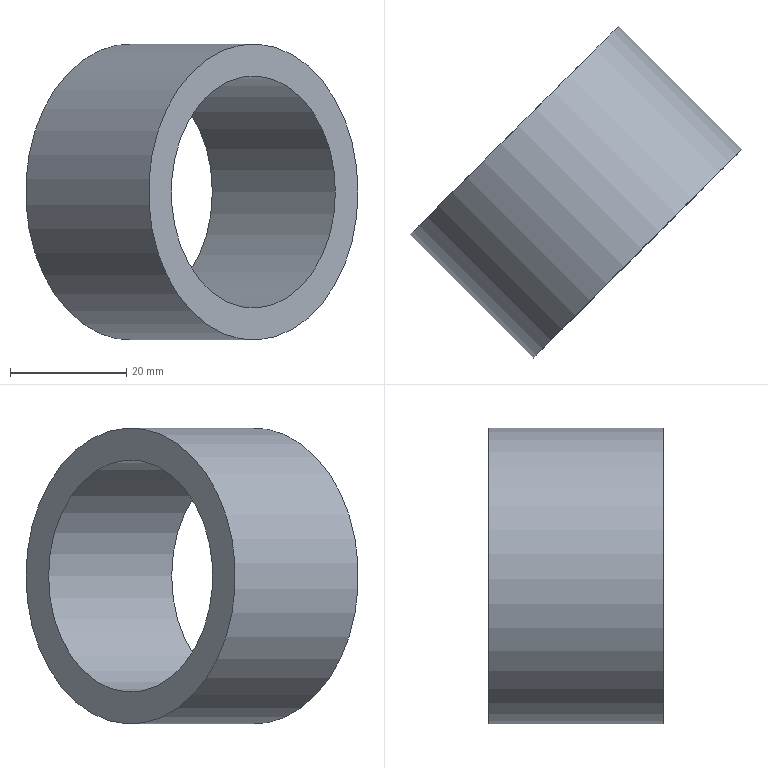Component | NX | CONN_FRAME_CONN_POST | 1 solid | 4 faces | box 57.28 x 57.28 x 51 mm | volume 23586 mm3 | cylinder 2 | plane 2 | commonest cylinder face diameters 51 x1 40 x1
STEP:
#1=CARTESIAN_POINT('',(0.,0.,0.));
#2=DIRECTION('',(0.,0.,1.));
#3=DIRECTION('',(1.,0.,0.));
#4=AXIS2_PLACEMENT_3D('',#1,#2,#3);
#5=CARTESIAN_POINT('',(-329.579,372.087,460.));
#6=VERTEX_POINT('',#5);
#7=CARTESIAN_POINT('',(-347.61,354.056,460.));
#8=DIRECTION('',(0.7071,-0.7071,0.));
#9=DIRECTION('',(0.7071,0.7071,0.));
#10=AXIS2_PLACEMENT_3D('',#7,#8,#9);
#11=CIRCLE('',#10,25.5);
#12=CARTESIAN_POINT('',(-347.61,354.056,460.));
#13=DIRECTION('',(0.7071,-0.7071,0.));
#14=DIRECTION('',(-0.7071,-0.7071,0.));
#15=AXIS2_PLACEMENT_3D('',#12,#13,#14);
#16=CYLINDRICAL_SURFACE('',#15,25.5);
#17=CARTESIAN_POINT('',(3.142,0.));
#18=DIRECTION('',(1.,0.));
#19=VECTOR('',#18,1.);
#20=LINE('',#17,#19);
#21=(GEOMETRIC_REPRESENTATION_CONTEXT(2)PARAMETRIC_REPRESENTATION_CONTEXT()REPRESENTATION_CONTEXT('',''));
#22=DEFINITIONAL_REPRESENTATION('',(#20),#21);
#23=PCURVE('',#16,#22);
#24=CARTESIAN_POINT('',(-347.61,354.056,460.));
#25=DIRECTION('',(0.7071,-0.7071,0.));
#26=DIRECTION('',(-0.7071,-0.7071,0.));
#27=AXIS2_PLACEMENT_3D('',#24,#25,#26);
#28=PLANE('',#27);
#29=CARTESIAN_POINT('',(0.,0.));
#30=DIRECTION('',(-1.,0.));
#31=AXIS2_PLACEMENT_2D('',#29,#30);
#32=CIRCLE('',#31,25.5);
#33=(GEOMETRIC_REPRESENTATION_CONTEXT(2)PARAMETRIC_REPRESENTATION_CONTEXT()REPRESENTATION_CONTEXT('',''));
#34=DEFINITIONAL_REPRESENTATION('',(#32),#33);
#35=PCURVE('',#28,#34);
#36=SURFACE_CURVE('',#11,(#23,#35),.PCURVE_S1.);
#37=EDGE_CURVE('',#6,#6,#36,.T.);
#38=ORIENTED_EDGE('',*,*,#37,.T.);
#39=CARTESIAN_POINT('',(-308.366,350.874,460.));
#40=VERTEX_POINT('',#39);
#41=CARTESIAN_POINT('',(-329.579,372.087,460.));
#42=CARTESIAN_POINT('',(-308.366,350.874,460.));
#43=B_SPLINE_CURVE_WITH_KNOTS('',1,(#41,#42),.UNSPECIFIED.,.F.,.F.,(2,2),(0.,30.),.PIECEWISE_BEZIER_KNOTS.);
#44=CARTESIAN_POINT('',(9.425,0.));
#45=DIRECTION('',(0.,1.));
#46=VECTOR('',#45,1.);
#47=LINE('',#44,#46);
#48=(GEOMETRIC_REPRESENTATION_CONTEXT(2)PARAMETRIC_REPRESENTATION_CONTEXT()REPRESENTATION_CONTEXT('',''));
#49=DEFINITIONAL_REPRESENTATION('',(#47),#48);
#50=PCURVE('',#16,#49);
#51=CARTESIAN_POINT('',(3.142,0.));
#52=DIRECTION('',(0.,1.));
#53=VECTOR('',#52,1.);
#54=LINE('',#51,#53);
#55=(GEOMETRIC_REPRESENTATION_CONTEXT(2)PARAMETRIC_REPRESENTATION_CONTEXT()REPRESENTATION_CONTEXT('',''));
#56=DEFINITIONAL_REPRESENTATION('',(#54),#55);
#57=PCURVE('',#16,#56);
#58=SEAM_CURVE('',#43,(#50,#57),.PCURVE_S1.);
#59=EDGE_CURVE('',#6,#40,#58,.T.);
#60=ORIENTED_EDGE('',*,*,#59,.T.);
#61=CARTESIAN_POINT('',(-326.397,332.843,460.));
#62=DIRECTION('',(0.7071,-0.7071,0.));
#63=DIRECTION('',(0.7071,0.7071,0.));
#64=AXIS2_PLACEMENT_3D('',#61,#62,#63);
#65=CIRCLE('',#64,25.5);
#66=CARTESIAN_POINT('',(3.142,30.));
#67=DIRECTION('',(1.,0.));
#68=VECTOR('',#67,1.);
#69=LINE('',#66,#68);
#70=(GEOMETRIC_REPRESENTATION_CONTEXT(2)PARAMETRIC_REPRESENTATION_CONTEXT()REPRESENTATION_CONTEXT('',''));
#71=DEFINITIONAL_REPRESENTATION('',(#69),#70);
#72=PCURVE('',#16,#71);
#73=CARTESIAN_POINT('',(-326.397,332.843,460.));
#74=DIRECTION('',(0.7071,-0.7071,0.));
#75=DIRECTION('',(-0.7071,-0.7071,0.));
#76=AXIS2_PLACEMENT_3D('',#73,#74,#75);
#77=PLANE('',#76);
#78=CARTESIAN_POINT('',(0.,0.));
#79=DIRECTION('',(-1.,0.));
#80=AXIS2_PLACEMENT_2D('',#78,#79);
#81=CIRCLE('',#80,25.5);
#82=(GEOMETRIC_REPRESENTATION_CONTEXT(2)PARAMETRIC_REPRESENTATION_CONTEXT()REPRESENTATION_CONTEXT('',''));
#83=DEFINITIONAL_REPRESENTATION('',(#81),#82);
#84=PCURVE('',#77,#83);
#85=SURFACE_CURVE('',#65,(#72,#84),.PCURVE_S1.);
#86=EDGE_CURVE('',#40,#40,#85,.T.);
#87=ORIENTED_EDGE('',*,*,#86,.F.);
#88=ORIENTED_EDGE('',*,*,#59,.F.);
#89=EDGE_LOOP('',(#38,#60,#87,#88));
#90=FACE_BOUND('',#89,.T.);
#91=ADVANCED_FACE('',(#90),#16,.T.);
#92=CARTESIAN_POINT('',(-333.468,368.198,460.));
#93=VERTEX_POINT('',#92);
#94=CARTESIAN_POINT('',(-347.61,354.056,460.));
#95=DIRECTION('',(0.7071,-0.7071,0.));
#96=DIRECTION('',(0.7071,0.7071,0.));
#97=AXIS2_PLACEMENT_3D('',#94,#95,#96);
#98=CIRCLE('',#97,20.);
#99=CARTESIAN_POINT('',(-347.61,354.056,460.));
#100=DIRECTION('',(0.7071,-0.7071,0.));
#101=DIRECTION('',(-0.7071,-0.7071,0.));
#102=AXIS2_PLACEMENT_3D('',#99,#100,#101);
#103=CYLINDRICAL_SURFACE('',#102,20.);
#104=CARTESIAN_POINT('',(3.142,0.));
#105=DIRECTION('',(1.,0.));
#106=VECTOR('',#105,1.);
#107=LINE('',#104,#106);
#108=(GEOMETRIC_REPRESENTATION_CONTEXT(2)PARAMETRIC_REPRESENTATION_CONTEXT()REPRESENTATION_CONTEXT('',''));
#109=DEFINITIONAL_REPRESENTATION('',(#107),#108);
#110=PCURVE('',#103,#109);
#111=CARTESIAN_POINT('',(0.,0.));
#112=DIRECTION('',(-1.,0.));
#113=AXIS2_PLACEMENT_2D('',#111,#112);
#114=CIRCLE('',#113,20.);
#115=(GEOMETRIC_REPRESENTATION_CONTEXT(2)PARAMETRIC_REPRESENTATION_CONTEXT()REPRESENTATION_CONTEXT('',''));
#116=DEFINITIONAL_REPRESENTATION('',(#114),#115);
#117=PCURVE('',#28,#116);
#118=SURFACE_CURVE('',#98,(#110,#117),.PCURVE_S1.);
#119=EDGE_CURVE('',#93,#93,#118,.T.);
#120=ORIENTED_EDGE('',*,*,#119,.T.);
#121=CARTESIAN_POINT('',(-312.255,346.985,460.));
#122=VERTEX_POINT('',#121);
#123=CARTESIAN_POINT('',(-333.468,368.198,460.));
#124=CARTESIAN_POINT('',(-312.255,346.985,460.));
#125=B_SPLINE_CURVE_WITH_KNOTS('',1,(#123,#124),.UNSPECIFIED.,.F.,.F.,(2,2),(0.,30.),.PIECEWISE_BEZIER_KNOTS.);
#126=CARTESIAN_POINT('',(9.425,0.));
#127=DIRECTION('',(0.,1.));
#128=VECTOR('',#127,1.);
#129=LINE('',#126,#128);
#130=(GEOMETRIC_REPRESENTATION_CONTEXT(2)PARAMETRIC_REPRESENTATION_CONTEXT()REPRESENTATION_CONTEXT('',''));
#131=DEFINITIONAL_REPRESENTATION('',(#129),#130);
#132=PCURVE('',#103,#131);
#133=CARTESIAN_POINT('',(3.142,0.));
#134=DIRECTION('',(0.,1.));
#135=VECTOR('',#134,1.);
#136=LINE('',#133,#135);
#137=(GEOMETRIC_REPRESENTATION_CONTEXT(2)PARAMETRIC_REPRESENTATION_CONTEXT()REPRESENTATION_CONTEXT('',''));
#138=DEFINITIONAL_REPRESENTATION('',(#136),#137);
#139=PCURVE('',#103,#138);
#140=SEAM_CURVE('',#125,(#132,#139),.PCURVE_S1.);
#141=EDGE_CURVE('',#93,#122,#140,.T.);
#142=ORIENTED_EDGE('',*,*,#141,.T.);
#143=CARTESIAN_POINT('',(-326.397,332.843,460.));
#144=DIRECTION('',(0.7071,-0.7071,0.));
#145=DIRECTION('',(0.7071,0.7071,0.));
#146=AXIS2_PLACEMENT_3D('',#143,#144,#145);
#147=CIRCLE('',#146,20.);
#148=CARTESIAN_POINT('',(3.142,30.));
#149=DIRECTION('',(1.,0.));
#150=VECTOR('',#149,1.);
#151=LINE('',#148,#150);
#152=(GEOMETRIC_REPRESENTATION_CONTEXT(2)PARAMETRIC_REPRESENTATION_CONTEXT()REPRESENTATION_CONTEXT('',''));
#153=DEFINITIONAL_REPRESENTATION('',(#151),#152);
#154=PCURVE('',#103,#153);
#155=CARTESIAN_POINT('',(0.,0.));
#156=DIRECTION('',(-1.,0.));
#157=AXIS2_PLACEMENT_2D('',#155,#156);
#158=CIRCLE('',#157,20.);
#159=(GEOMETRIC_REPRESENTATION_CONTEXT(2)PARAMETRIC_REPRESENTATION_CONTEXT()REPRESENTATION_CONTEXT('',''));
#160=DEFINITIONAL_REPRESENTATION('',(#158),#159);
#161=PCURVE('',#77,#160);
#162=SURFACE_CURVE('',#147,(#154,#161),.PCURVE_S1.);
#163=EDGE_CURVE('',#122,#122,#162,.T.);
#164=ORIENTED_EDGE('',*,*,#163,.F.);
#165=ORIENTED_EDGE('',*,*,#141,.F.);
#166=EDGE_LOOP('',(#120,#142,#164,#165));
#167=FACE_BOUND('',#166,.F.);
#168=ADVANCED_FACE('',(#167),#103,.F.);
#169=ORIENTED_EDGE('',*,*,#37,.F.);
#170=EDGE_LOOP('',(#169));
#171=FACE_BOUND('',#170,.T.);
#172=ORIENTED_EDGE('',*,*,#119,.T.);
#173=EDGE_LOOP('',(#172));
#174=FACE_BOUND('',#173,.T.);
#175=ADVANCED_FACE('',(#171,#174),#28,.F.);
#176=ORIENTED_EDGE('',*,*,#86,.T.);
#177=EDGE_LOOP('',(#176));
#178=FACE_BOUND('',#177,.T.);
#179=ORIENTED_EDGE('',*,*,#163,.F.);
#180=EDGE_LOOP('',(#179));
#181=FACE_BOUND('',#180,.T.);
#182=ADVANCED_FACE('',(#178,#181),#77,.T.);
#183=CLOSED_SHELL('',(#91,#168,#175,#182));
#184=MANIFOLD_SOLID_BREP('',#183);
#185=(LENGTH_UNIT()NAMED_UNIT(*)SI_UNIT(.MILLI.,.METRE.));
#186=UNCERTAINTY_MEASURE_WITH_UNIT(LENGTH_MEASURE(0.00001),#185,'','');
#187=(NAMED_UNIT(*)PLANE_ANGLE_UNIT()SI_UNIT($,.RADIAN.));
#188=(NAMED_UNIT(*)SI_UNIT($,.STERADIAN.)SOLID_ANGLE_UNIT());
#189=(GEOMETRIC_REPRESENTATION_CONTEXT(3)GLOBAL_UNCERTAINTY_ASSIGNED_CONTEXT((#186))GLOBAL_UNIT_ASSIGNED_CONTEXT((#185,#187,#188))REPRESENTATION_CONTEXT('',''));
#190=ADVANCED_BREP_SHAPE_REPRESENTATION('',(#4,#184),#189);